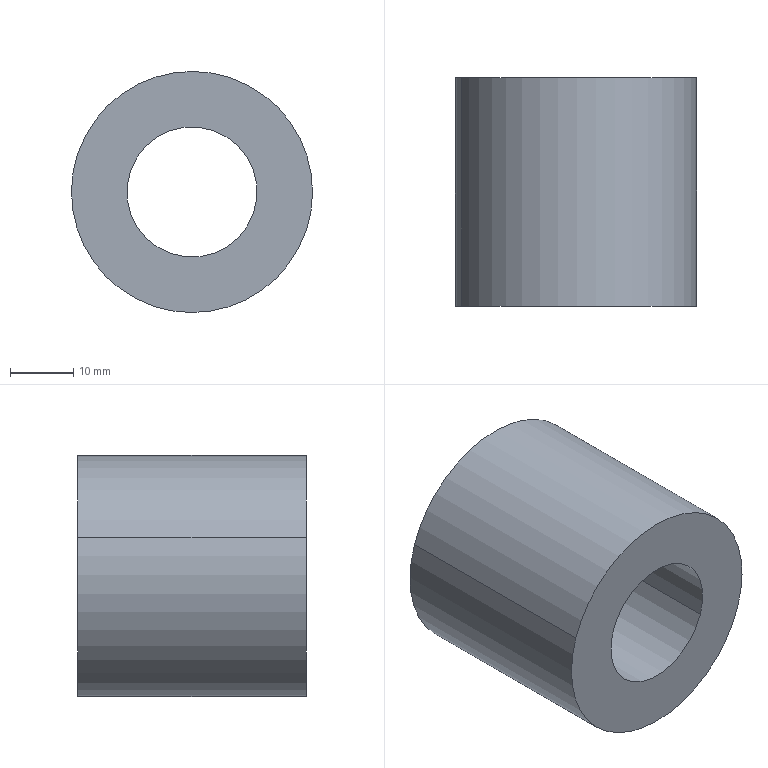Component | SolidWorks | HolePunchingCouplingBushing-1 | 1 solid | 6 faces | box 38 x 36 x 38 mm | volume 28946 mm3 | cylinder 4 | plane 2 | commonest cylinder face diameters 20.5 x2 38 x2
build123d program:
from build123d import *

# Parameters (mm, degrees)
SKETCH1_R      = 19
SKETCH1_R_2    = 10.25
EXTRUDE1_DEPTH = 36


with BuildPart() as part:
    # Sketch1 → Extrude1 (new body)
    with BuildSketch(Plane.XY):
        Circle(SKETCH1_R)
        Circle(SKETCH1_R_2, mode=Mode.SUBTRACT)
    extrude(amount=EXTRUDE1_DEPTH)


solid = part.part

# Placed as in the assembly
solid = solid.moved(Location((-164.784, 351.983, 4), (90, 0, 0)))
STEP:
#1=COLOUR_RGB('',0.7922,0.8196,0.9333);
#2=FILL_AREA_STYLE_COLOUR('',#1);
#3=FILL_AREA_STYLE('',(#2));
#4=SURFACE_STYLE_FILL_AREA(#3);
#5=SURFACE_SIDE_STYLE('',(#4));
#6=SURFACE_STYLE_USAGE(.BOTH.,#5);
#7=PRESENTATION_STYLE_ASSIGNMENT((#6));
#8=CARTESIAN_POINT('',(-6.87,13.858,0.2864));
#9=VERTEX_POINT('',#8);
#10=CARTESIAN_POINT('',(-6.105,13.858,0.02854));
#11=VERTEX_POINT('',#10);
#12=CARTESIAN_POINT('',(-6.488,13.858,0.1575));
#13=DIRECTION('',(-0.,1.,-0.));
#14=DIRECTION('',(0.9476,0.,-0.3195));
#15=AXIS2_PLACEMENT_3D('',#12,#13,#14);
#16=CIRCLE('',#15,0.4035);
#17=EDGE_CURVE('',#9,#11,#16,.T.);
#18=ORIENTED_EDGE('',*,*,#17,.T.);
#19=CARTESIAN_POINT('',(-6.105,12.44,0.02854));
#20=VERTEX_POINT('',#19);
#21=CARTESIAN_POINT('',(-6.105,13.858,0.02854));
#22=DIRECTION('',(0.,-1.,0.));
#23=VECTOR('',#22,39.37);
#24=LINE('',#21,#23);
#25=EDGE_CURVE('',#11,#20,#24,.T.);
#26=ORIENTED_EDGE('',*,*,#25,.T.);
#27=CARTESIAN_POINT('',(-6.87,12.44,0.2864));
#28=VERTEX_POINT('',#27);
#29=CARTESIAN_POINT('',(-6.488,12.44,0.1575));
#30=DIRECTION('',(-0.,1.,-0.));
#31=DIRECTION('',(0.9476,0.,-0.3195));
#32=AXIS2_PLACEMENT_3D('',#29,#30,#31);
#33=CIRCLE('',#32,0.4035);
#34=EDGE_CURVE('',#28,#20,#33,.T.);
#35=ORIENTED_EDGE('',*,*,#34,.F.);
#36=CARTESIAN_POINT('',(-6.87,13.858,0.2864));
#37=DIRECTION('',(0.,-1.,0.));
#38=VECTOR('',#37,39.37);
#39=LINE('',#36,#38);
#40=EDGE_CURVE('',#9,#28,#39,.T.);
#41=ORIENTED_EDGE('',*,*,#40,.F.);
#42=EDGE_LOOP('',(#18,#26,#35,#41));
#43=FACE_OUTER_BOUND('',#42,.T.);
#44=CARTESIAN_POINT('',(-6.488,13.858,0.1575));
#45=DIRECTION('',(0.,-1.,0.));
#46=DIRECTION('',(-0.9476,0.,0.3195));
#47=AXIS2_PLACEMENT_3D('',#44,#45,#46);
#48=CYLINDRICAL_SURFACE('',#47,0.4035);
#49=ADVANCED_FACE('',(#43),#48,.F.);
#50=CARTESIAN_POINT('',(-5.779,13.858,-0.08153));
#51=VERTEX_POINT('',#50);
#52=CARTESIAN_POINT('',(-7.196,13.858,0.3965));
#53=VERTEX_POINT('',#52);
#54=CARTESIAN_POINT('',(-6.488,13.858,0.1575));
#55=DIRECTION('',(-0.,1.,-0.));
#56=DIRECTION('',(0.9476,0.,-0.3195));
#57=AXIS2_PLACEMENT_3D('',#54,#55,#56);
#58=CIRCLE('',#57,0.748);
#59=EDGE_CURVE('',#51,#53,#58,.T.);
#60=ORIENTED_EDGE('',*,*,#59,.F.);
#61=CARTESIAN_POINT('',(-5.779,12.44,-0.08153));
#62=VERTEX_POINT('',#61);
#63=CARTESIAN_POINT('',(-5.779,13.858,-0.08153));
#64=DIRECTION('',(0.,-1.,0.));
#65=VECTOR('',#64,39.37);
#66=LINE('',#63,#65);
#67=EDGE_CURVE('',#51,#62,#66,.T.);
#68=ORIENTED_EDGE('',*,*,#67,.T.);
#69=CARTESIAN_POINT('',(-7.196,12.44,0.3965));
#70=VERTEX_POINT('',#69);
#71=CARTESIAN_POINT('',(-6.488,12.44,0.1575));
#72=DIRECTION('',(-0.,1.,-0.));
#73=DIRECTION('',(0.9476,0.,-0.3195));
#74=AXIS2_PLACEMENT_3D('',#71,#72,#73);
#75=CIRCLE('',#74,0.748);
#76=EDGE_CURVE('',#62,#70,#75,.T.);
#77=ORIENTED_EDGE('',*,*,#76,.T.);
#78=CARTESIAN_POINT('',(-7.196,13.858,0.3965));
#79=DIRECTION('',(0.,-1.,0.));
#80=VECTOR('',#79,39.37);
#81=LINE('',#78,#80);
#82=EDGE_CURVE('',#53,#70,#81,.T.);
#83=ORIENTED_EDGE('',*,*,#82,.F.);
#84=EDGE_LOOP('',(#60,#68,#77,#83));
#85=FACE_OUTER_BOUND('',#84,.T.);
#86=CARTESIAN_POINT('',(-6.488,13.858,0.1575));
#87=DIRECTION('',(0.,-1.,0.));
#88=DIRECTION('',(-0.9476,0.,0.3195));
#89=AXIS2_PLACEMENT_3D('',#86,#87,#88);
#90=CYLINDRICAL_SURFACE('',#89,0.748);
#91=ADVANCED_FACE('',(#85),#90,.T.);
#92=CARTESIAN_POINT('',(-6.488,13.858,0.1575));
#93=DIRECTION('',(-0.,1.,-0.));
#94=DIRECTION('',(0.9476,0.,-0.3195));
#95=AXIS2_PLACEMENT_3D('',#92,#93,#94);
#96=CIRCLE('',#95,0.748);
#97=EDGE_CURVE('',#53,#51,#96,.T.);
#98=ORIENTED_EDGE('',*,*,#97,.T.);
#99=ORIENTED_EDGE('',*,*,#59,.T.);
#100=EDGE_LOOP('',(#98,#99));
#101=FACE_OUTER_BOUND('',#100,.T.);
#102=ORIENTED_EDGE('',*,*,#17,.F.);
#103=CARTESIAN_POINT('',(-6.488,13.858,0.1575));
#104=DIRECTION('',(-0.,1.,-0.));
#105=DIRECTION('',(0.9476,0.,-0.3195));
#106=AXIS2_PLACEMENT_3D('',#103,#104,#105);
#107=CIRCLE('',#106,0.4035);
#108=EDGE_CURVE('',#11,#9,#107,.T.);
#109=ORIENTED_EDGE('',*,*,#108,.F.);
#110=EDGE_LOOP('',(#102,#109));
#111=FACE_BOUND('',#110,.T.);
#112=CARTESIAN_POINT('',(-6.488,13.858,0.1575));
#113=DIRECTION('',(-0.,1.,-0.));
#114=DIRECTION('',(0.9476,0.,-0.3195));
#115=AXIS2_PLACEMENT_3D('',#112,#113,#114);
#116=PLANE('',#115);
#117=ADVANCED_FACE('',(#101,#111),#116,.T.);
#118=CARTESIAN_POINT('',(-6.488,12.44,0.1575));
#119=DIRECTION('',(-0.,1.,-0.));
#120=DIRECTION('',(0.9476,0.,-0.3195));
#121=AXIS2_PLACEMENT_3D('',#118,#119,#120);
#122=CIRCLE('',#121,0.748);
#123=EDGE_CURVE('',#70,#62,#122,.T.);
#124=ORIENTED_EDGE('',*,*,#123,.F.);
#125=ORIENTED_EDGE('',*,*,#76,.F.);
#126=EDGE_LOOP('',(#124,#125));
#127=FACE_OUTER_BOUND('',#126,.T.);
#128=ORIENTED_EDGE('',*,*,#34,.T.);
#129=CARTESIAN_POINT('',(-6.488,12.44,0.1575));
#130=DIRECTION('',(-0.,1.,-0.));
#131=DIRECTION('',(0.9476,0.,-0.3195));
#132=AXIS2_PLACEMENT_3D('',#129,#130,#131);
#133=CIRCLE('',#132,0.4035);
#134=EDGE_CURVE('',#20,#28,#133,.T.);
#135=ORIENTED_EDGE('',*,*,#134,.T.);
#136=EDGE_LOOP('',(#128,#135));
#137=FACE_BOUND('',#136,.T.);
#138=CARTESIAN_POINT('',(-6.488,12.44,0.1575));
#139=DIRECTION('',(-0.,1.,-0.));
#140=DIRECTION('',(0.9476,0.,-0.3195));
#141=AXIS2_PLACEMENT_3D('',#138,#139,#140);
#142=PLANE('',#141);
#143=ADVANCED_FACE('',(#127,#137),#142,.F.);
#144=ORIENTED_EDGE('',*,*,#67,.F.);
#145=ORIENTED_EDGE('',*,*,#97,.F.);
#146=ORIENTED_EDGE('',*,*,#82,.T.);
#147=ORIENTED_EDGE('',*,*,#123,.T.);
#148=EDGE_LOOP('',(#144,#145,#146,#147));
#149=FACE_OUTER_BOUND('',#148,.T.);
#150=CARTESIAN_POINT('',(-6.488,13.858,0.1575));
#151=DIRECTION('',(0.,-1.,0.));
#152=DIRECTION('',(-0.9476,0.,0.3195));
#153=AXIS2_PLACEMENT_3D('',#150,#151,#152);
#154=CYLINDRICAL_SURFACE('',#153,0.748);
#155=ADVANCED_FACE('',(#149),#154,.T.);
#156=ORIENTED_EDGE('',*,*,#25,.F.);
#157=ORIENTED_EDGE('',*,*,#108,.T.);
#158=ORIENTED_EDGE('',*,*,#40,.T.);
#159=ORIENTED_EDGE('',*,*,#134,.F.);
#160=EDGE_LOOP('',(#156,#157,#158,#159));
#161=FACE_OUTER_BOUND('',#160,.T.);
#162=CARTESIAN_POINT('',(-6.488,13.858,0.1575));
#163=DIRECTION('',(0.,-1.,0.));
#164=DIRECTION('',(-0.9476,0.,0.3195));
#165=AXIS2_PLACEMENT_3D('',#162,#163,#164);
#166=CYLINDRICAL_SURFACE('',#165,0.4035);
#167=ADVANCED_FACE('',(#161),#166,.F.);
#168=CLOSED_SHELL('',(#49,#91,#117,#143,#155,#167));
#169=MANIFOLD_SOLID_BREP('',#168);
#170=STYLED_ITEM('',(#7),#169);
#171=PRESENTATION_LAYER_ASSIGNMENT('','',(#170));
#172=CARTESIAN_POINT('',(0.,0.,0.));
#173=DIRECTION('',(0.,0.,1.));
#174=DIRECTION('',(1.,0.,0.));
#175=AXIS2_PLACEMENT_3D('',#172,#173,#174);
#176=(LENGTH_UNIT()NAMED_UNIT(*)SI_UNIT($,.METRE.));
#177=LENGTH_MEASURE_WITH_UNIT(LENGTH_MEASURE(0.0254),#176);
#178=DIMENSIONAL_EXPONENTS(1.,0.,0.,0.,0.,0.,0.);
#179=(CONVERSION_BASED_UNIT('',#177)LENGTH_UNIT()NAMED_UNIT(#178));
#180=UNCERTAINTY_MEASURE_WITH_UNIT(LENGTH_MEASURE(0.00001),#179,'','');
#181=(NAMED_UNIT(*)PLANE_ANGLE_UNIT()SI_UNIT($,.RADIAN.));
#182=(NAMED_UNIT(*)SI_UNIT($,.STERADIAN.)SOLID_ANGLE_UNIT());
#183=(GEOMETRIC_REPRESENTATION_CONTEXT(3)GLOBAL_UNCERTAINTY_ASSIGNED_CONTEXT((#180))GLOBAL_UNIT_ASSIGNED_CONTEXT((#179,#181,#182))REPRESENTATION_CONTEXT('',''));
#184=ADVANCED_BREP_SHAPE_REPRESENTATION('',(#169,#175),#183);
#185=(LENGTH_UNIT()NAMED_UNIT(*)SI_UNIT($,.METRE.));
#186=LENGTH_MEASURE_WITH_UNIT(LENGTH_MEASURE(0.0254),#185);
#187=DIMENSIONAL_EXPONENTS(1.,0.,0.,0.,0.,0.,0.);
#188=(CONVERSION_BASED_UNIT('',#186)LENGTH_UNIT()NAMED_UNIT(#187));
#189=UNCERTAINTY_MEASURE_WITH_UNIT(LENGTH_MEASURE(0.00001),#188,'','');
#190=(NAMED_UNIT(*)PLANE_ANGLE_UNIT()SI_UNIT($,.RADIAN.));
#191=(NAMED_UNIT(*)SI_UNIT($,.STERADIAN.)SOLID_ANGLE_UNIT());
#192=(GEOMETRIC_REPRESENTATION_CONTEXT(3)GLOBAL_UNCERTAINTY_ASSIGNED_CONTEXT((#189))GLOBAL_UNIT_ASSIGNED_CONTEXT((#188,#190,#191))REPRESENTATION_CONTEXT('',''));
#193=MECHANICAL_DESIGN_GEOMETRIC_PRESENTATION_REPRESENTATION('',(#170),#192);